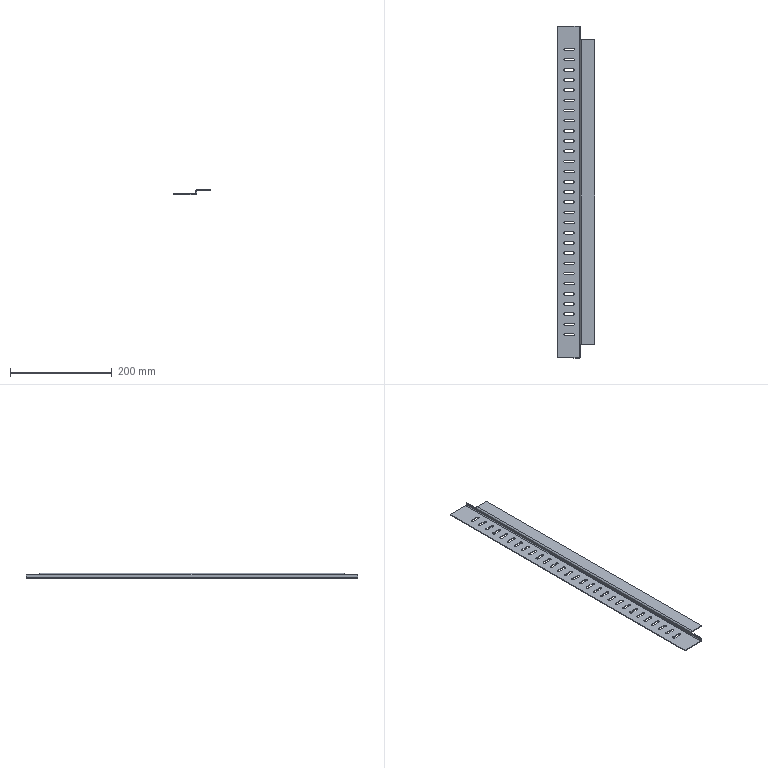Component | SolidWorks | TopCoverAssembly-1_TopCoverLeftAndRightFlange-2 | 1 solid | 169 faces | volume 71798 mm3 | cylinder 91 | plane 78 | commonest cylinder face diameters 5 x87 6 x2 3 x2